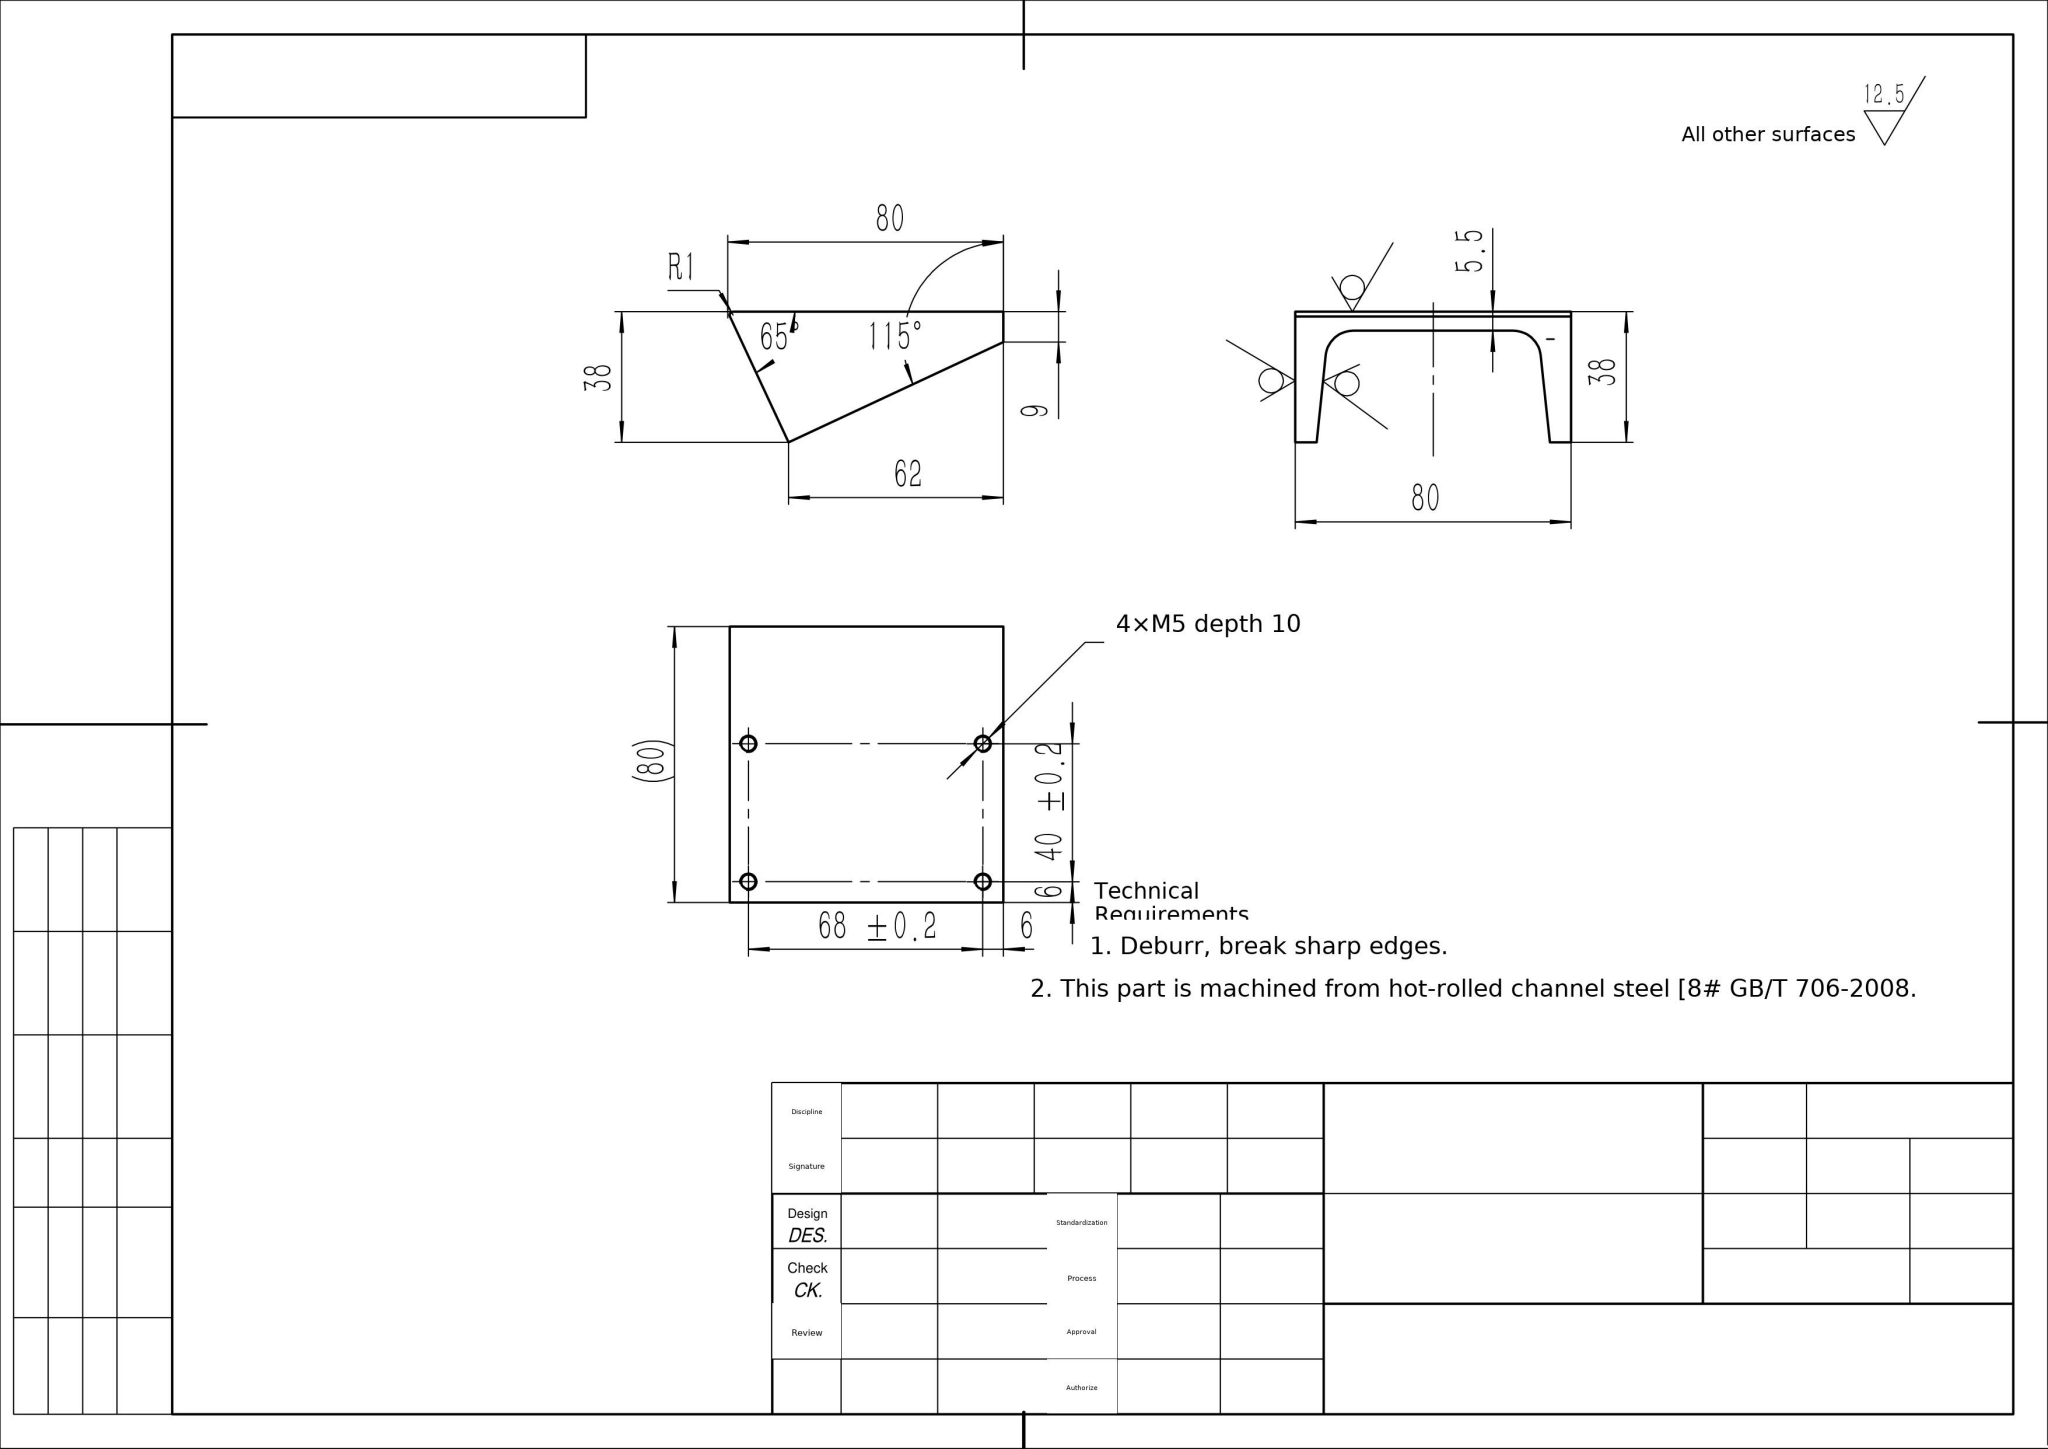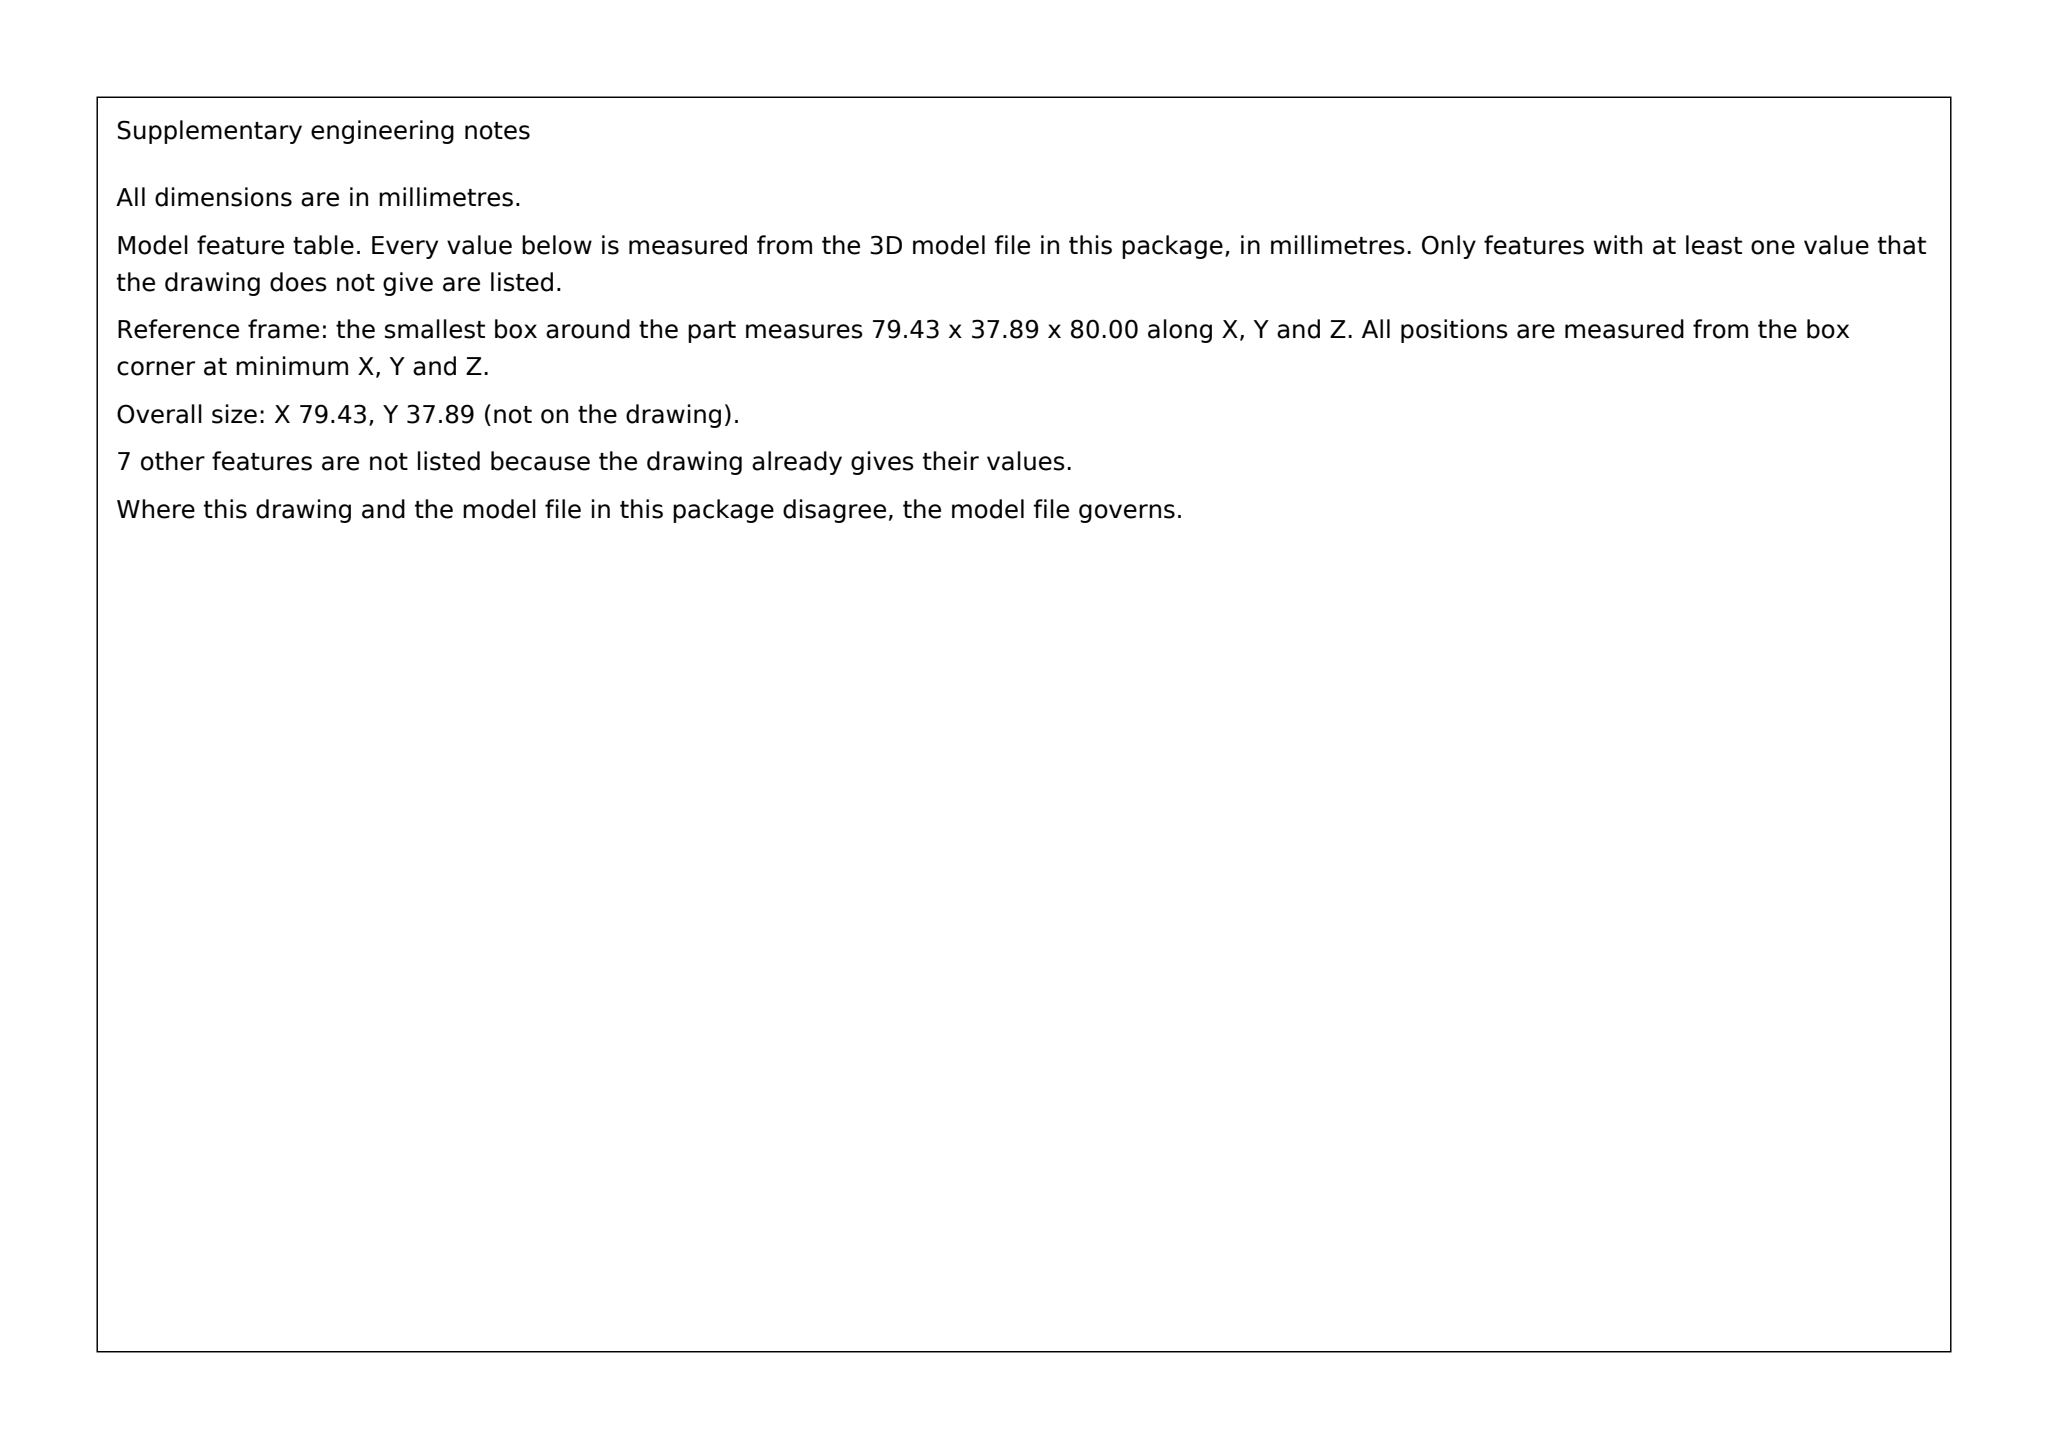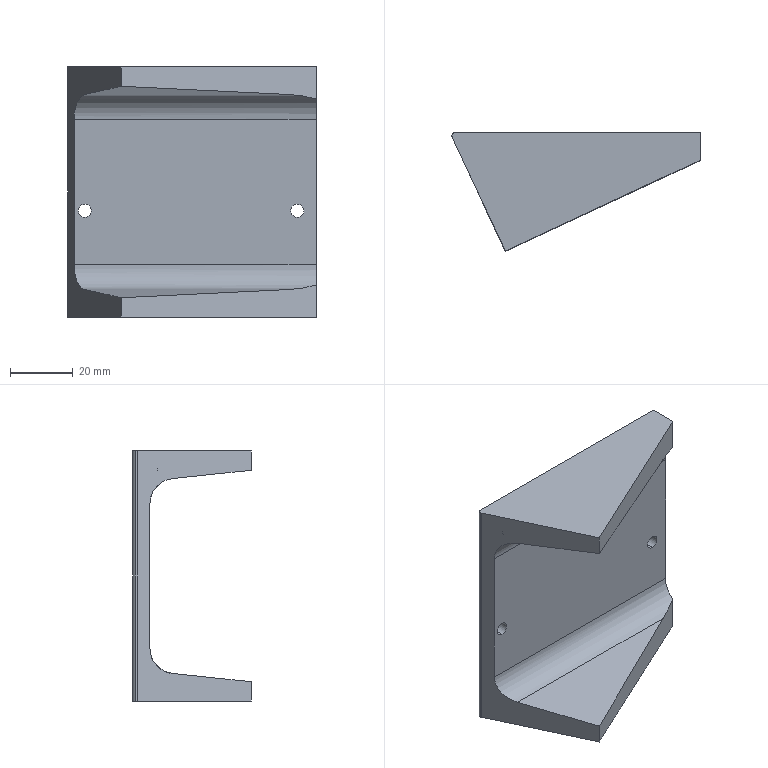Part | SolidWorks | mm | material hot-rolled channel steel [8# GB/T 706-2008 | 1 solid | 24 faces | box 79.43 x 37.89 x 80 mm | volume 58753 mm3 | cylinder 12 | plane 12 | commonest cylinder face diameters 4.2 x8 2 x2 16 x2
STEP:
#1=CARTESIAN_POINT('',(-79.43,-1.,80.));
#2=VERTEX_POINT('',#1);
#3=CARTESIAN_POINT('',(-79.337,-1.423,80.));
#4=VERTEX_POINT('',#3);
#5=CARTESIAN_POINT('',(-78.43,-1.,80.));
#6=DIRECTION('',(0.,-0.,1.));
#7=DIRECTION('',(0.,1.,0.));
#8=AXIS2_PLACEMENT_3D('',#5,#6,#7);
#9=CIRCLE('',#8,1.);
#10=EDGE_CURVE('',#2,#4,#9,.T.);
#11=ORIENTED_EDGE('',*,*,#10,.F.);
#12=CARTESIAN_POINT('',(-79.43,-1.,0.));
#13=VERTEX_POINT('',#12);
#14=CARTESIAN_POINT('',(-79.43,-1.,80.));
#15=DIRECTION('',(0.,0.,-1.));
#16=VECTOR('',#15,1000.);
#17=LINE('',#14,#16);
#18=EDGE_CURVE('',#2,#13,#17,.T.);
#19=ORIENTED_EDGE('',*,*,#18,.T.);
#20=CARTESIAN_POINT('',(-79.337,-1.423,0.));
#21=VERTEX_POINT('',#20);
#22=CARTESIAN_POINT('',(-78.43,-1.,0.));
#23=DIRECTION('',(0.,0.,-1.));
#24=DIRECTION('',(1.,0.,0.));
#25=AXIS2_PLACEMENT_3D('',#22,#23,#24);
#26=CIRCLE('',#25,1.);
#27=EDGE_CURVE('',#21,#13,#26,.T.);
#28=ORIENTED_EDGE('',*,*,#27,.F.);
#29=CARTESIAN_POINT('',(-79.337,-1.423,80.));
#30=DIRECTION('',(0.,0.,-1.));
#31=VECTOR('',#30,1000.);
#32=LINE('',#29,#31);
#33=EDGE_CURVE('',#4,#21,#32,.T.);
#34=ORIENTED_EDGE('',*,*,#33,.F.);
#35=EDGE_LOOP('',(#11,#19,#28,#34));
#36=FACE_OUTER_BOUND('',#35,.T.);
#37=CARTESIAN_POINT('',(-78.43,-1.,80.));
#38=DIRECTION('',(0.,0.,-1.));
#39=DIRECTION('',(-1.,0.,0.));
#40=AXIS2_PLACEMENT_3D('',#37,#38,#39);
#41=CYLINDRICAL_SURFACE('',#40,1.);
#42=ADVANCED_FACE('',(#36),#41,.T.);
#43=CARTESIAN_POINT('',(-6.,-5.5,31.9));
#44=VERTEX_POINT('',#43);
#45=CARTESIAN_POINT('',(-6.,-5.5,36.1));
#46=VERTEX_POINT('',#45);
#47=CARTESIAN_POINT('',(-6.,-5.5,34.));
#48=DIRECTION('',(-0.,1.,0.));
#49=DIRECTION('',(-1.,0.,0.));
#50=AXIS2_PLACEMENT_3D('',#47,#48,#49);
#51=CIRCLE('',#50,2.1);
#52=EDGE_CURVE('',#44,#46,#51,.T.);
#53=ORIENTED_EDGE('',*,*,#52,.F.);
#54=CARTESIAN_POINT('',(-6.,-0.,31.9));
#55=VERTEX_POINT('',#54);
#56=CARTESIAN_POINT('',(-6.,-0.,31.9));
#57=DIRECTION('',(0.,1.,0.));
#58=VECTOR('',#57,1000.);
#59=LINE('',#56,#58);
#60=EDGE_CURVE('',#44,#55,#59,.T.);
#61=ORIENTED_EDGE('',*,*,#60,.T.);
#62=CARTESIAN_POINT('',(-6.,-0.,36.1));
#63=VERTEX_POINT('',#62);
#64=CARTESIAN_POINT('',(-6.,-0.,34.));
#65=DIRECTION('',(0.,1.,0.));
#66=DIRECTION('',(0.,0.,1.));
#67=AXIS2_PLACEMENT_3D('',#64,#65,#66);
#68=CIRCLE('',#67,2.1);
#69=EDGE_CURVE('',#55,#63,#68,.T.);
#70=ORIENTED_EDGE('',*,*,#69,.T.);
#71=CARTESIAN_POINT('',(-6.,-0.,36.1));
#72=DIRECTION('',(0.,1.,0.));
#73=VECTOR('',#72,1000.);
#74=LINE('',#71,#73);
#75=EDGE_CURVE('',#46,#63,#74,.T.);
#76=ORIENTED_EDGE('',*,*,#75,.F.);
#77=EDGE_LOOP('',(#53,#61,#70,#76));
#78=FACE_OUTER_BOUND('',#77,.T.);
#79=CARTESIAN_POINT('',(-6.,-0.,34.));
#80=DIRECTION('',(0.,1.,0.));
#81=DIRECTION('',(0.,0.,1.));
#82=AXIS2_PLACEMENT_3D('',#79,#80,#81);
#83=CYLINDRICAL_SURFACE('',#82,2.1);
#84=ADVANCED_FACE('',(#78),#83,.F.);
#85=CARTESIAN_POINT('',(-6.,-8.,71.9));
#86=VERTEX_POINT('',#85);
#87=CARTESIAN_POINT('',(-6.,-8.,76.1));
#88=VERTEX_POINT('',#87);
#89=CARTESIAN_POINT('',(-6.,-8.,74.));
#90=DIRECTION('',(0.,1.,0.));
#91=DIRECTION('',(0.,0.,1.));
#92=AXIS2_PLACEMENT_3D('',#89,#90,#91);
#93=CIRCLE('',#92,2.1);
#94=EDGE_CURVE('',#86,#88,#93,.T.);
#95=ORIENTED_EDGE('',*,*,#94,.F.);
#96=CARTESIAN_POINT('',(-6.,-0.,71.9));
#97=VERTEX_POINT('',#96);
#98=CARTESIAN_POINT('',(-6.,-0.,71.9));
#99=DIRECTION('',(0.,1.,0.));
#100=VECTOR('',#99,1000.);
#101=LINE('',#98,#100);
#102=EDGE_CURVE('',#86,#97,#101,.T.);
#103=ORIENTED_EDGE('',*,*,#102,.T.);
#104=CARTESIAN_POINT('',(-6.,-0.,76.1));
#105=VERTEX_POINT('',#104);
#106=CARTESIAN_POINT('',(-6.,-0.,74.));
#107=DIRECTION('',(0.,1.,0.));
#108=DIRECTION('',(0.,0.,1.));
#109=AXIS2_PLACEMENT_3D('',#106,#107,#108);
#110=CIRCLE('',#109,2.1);
#111=EDGE_CURVE('',#97,#105,#110,.T.);
#112=ORIENTED_EDGE('',*,*,#111,.T.);
#113=CARTESIAN_POINT('',(-6.,-0.,76.1));
#114=DIRECTION('',(0.,1.,0.));
#115=VECTOR('',#114,1000.);
#116=LINE('',#113,#115);
#117=EDGE_CURVE('',#88,#105,#116,.T.);
#118=ORIENTED_EDGE('',*,*,#117,.F.);
#119=EDGE_LOOP('',(#95,#103,#112,#118));
#120=FACE_OUTER_BOUND('',#119,.T.);
#121=CARTESIAN_POINT('',(-6.,-0.,74.));
#122=DIRECTION('',(0.,1.,0.));
#123=DIRECTION('',(0.,0.,1.));
#124=AXIS2_PLACEMENT_3D('',#121,#122,#123);
#125=CYLINDRICAL_SURFACE('',#124,2.1);
#126=ADVANCED_FACE('',(#120),#125,.F.);
#127=CARTESIAN_POINT('',(-74.,-8.,71.9));
#128=VERTEX_POINT('',#127);
#129=CARTESIAN_POINT('',(-74.,-8.,76.1));
#130=VERTEX_POINT('',#129);
#131=CARTESIAN_POINT('',(-74.,-8.,74.));
#132=DIRECTION('',(0.,1.,0.));
#133=DIRECTION('',(0.,0.,1.));
#134=AXIS2_PLACEMENT_3D('',#131,#132,#133);
#135=CIRCLE('',#134,2.1);
#136=EDGE_CURVE('',#128,#130,#135,.T.);
#137=ORIENTED_EDGE('',*,*,#136,.F.);
#138=CARTESIAN_POINT('',(-74.,-0.,71.9));
#139=VERTEX_POINT('',#138);
#140=CARTESIAN_POINT('',(-74.,-0.,71.9));
#141=DIRECTION('',(0.,1.,0.));
#142=VECTOR('',#141,1000.);
#143=LINE('',#140,#142);
#144=EDGE_CURVE('',#128,#139,#143,.T.);
#145=ORIENTED_EDGE('',*,*,#144,.T.);
#146=CARTESIAN_POINT('',(-74.,-0.,76.1));
#147=VERTEX_POINT('',#146);
#148=CARTESIAN_POINT('',(-74.,-0.,74.));
#149=DIRECTION('',(0.,1.,0.));
#150=DIRECTION('',(0.,0.,1.));
#151=AXIS2_PLACEMENT_3D('',#148,#149,#150);
#152=CIRCLE('',#151,2.1);
#153=EDGE_CURVE('',#139,#147,#152,.T.);
#154=ORIENTED_EDGE('',*,*,#153,.T.);
#155=CARTESIAN_POINT('',(-74.,-0.,76.1));
#156=DIRECTION('',(0.,1.,0.));
#157=VECTOR('',#156,1000.);
#158=LINE('',#155,#157);
#159=EDGE_CURVE('',#130,#147,#158,.T.);
#160=ORIENTED_EDGE('',*,*,#159,.F.);
#161=EDGE_LOOP('',(#137,#145,#154,#160));
#162=FACE_OUTER_BOUND('',#161,.T.);
#163=CARTESIAN_POINT('',(-74.,-0.,74.));
#164=DIRECTION('',(0.,1.,0.));
#165=DIRECTION('',(0.,0.,1.));
#166=AXIS2_PLACEMENT_3D('',#163,#164,#165);
#167=CYLINDRICAL_SURFACE('',#166,2.1);
#168=ADVANCED_FACE('',(#162),#167,.F.);
#169=CARTESIAN_POINT('',(-74.,-5.5,31.9));
#170=VERTEX_POINT('',#169);
#171=CARTESIAN_POINT('',(-74.,-5.5,36.1));
#172=VERTEX_POINT('',#171);
#173=CARTESIAN_POINT('',(-74.,-5.5,34.));
#174=DIRECTION('',(-0.,1.,0.));
#175=DIRECTION('',(-1.,0.,0.));
#176=AXIS2_PLACEMENT_3D('',#173,#174,#175);
#177=CIRCLE('',#176,2.1);
#178=EDGE_CURVE('',#170,#172,#177,.T.);
#179=ORIENTED_EDGE('',*,*,#178,.F.);
#180=CARTESIAN_POINT('',(-74.,-0.,31.9));
#181=VERTEX_POINT('',#180);
#182=CARTESIAN_POINT('',(-74.,-0.,31.9));
#183=DIRECTION('',(0.,1.,0.));
#184=VECTOR('',#183,1000.);
#185=LINE('',#182,#184);
#186=EDGE_CURVE('',#170,#181,#185,.T.);
#187=ORIENTED_EDGE('',*,*,#186,.T.);
#188=CARTESIAN_POINT('',(-74.,-0.,36.1));
#189=VERTEX_POINT('',#188);
#190=CARTESIAN_POINT('',(-74.,-0.,34.));
#191=DIRECTION('',(0.,1.,0.));
#192=DIRECTION('',(0.,0.,1.));
#193=AXIS2_PLACEMENT_3D('',#190,#191,#192);
#194=CIRCLE('',#193,2.1);
#195=EDGE_CURVE('',#181,#189,#194,.T.);
#196=ORIENTED_EDGE('',*,*,#195,.T.);
#197=CARTESIAN_POINT('',(-74.,-0.,36.1));
#198=DIRECTION('',(0.,1.,0.));
#199=VECTOR('',#198,1000.);
#200=LINE('',#197,#199);
#201=EDGE_CURVE('',#172,#189,#200,.T.);
#202=ORIENTED_EDGE('',*,*,#201,.F.);
#203=EDGE_LOOP('',(#179,#187,#196,#202));
#204=FACE_OUTER_BOUND('',#203,.T.);
#205=CARTESIAN_POINT('',(-74.,-0.,34.));
#206=DIRECTION('',(0.,1.,0.));
#207=DIRECTION('',(0.,0.,1.));
#208=AXIS2_PLACEMENT_3D('',#205,#206,#207);
#209=CYLINDRICAL_SURFACE('',#208,2.1);
#210=ADVANCED_FACE('',(#204),#209,.F.);
#211=CARTESIAN_POINT('',(-78.43,-0.,80.));
#212=VERTEX_POINT('',#211);
#213=CARTESIAN_POINT('',(0.,0.,80.));
#214=VERTEX_POINT('',#213);
#215=CARTESIAN_POINT('',(-80.,-0.,80.));
#216=DIRECTION('',(1.,0.,0.));
#217=VECTOR('',#216,1000.);
#218=LINE('',#215,#217);
#219=EDGE_CURVE('',#212,#214,#218,.T.);
#220=ORIENTED_EDGE('',*,*,#219,.F.);
#221=CARTESIAN_POINT('',(-78.43,-1.,80.));
#222=DIRECTION('',(0.,-0.,1.));
#223=DIRECTION('',(0.,1.,0.));
#224=AXIS2_PLACEMENT_3D('',#221,#222,#223);
#225=CIRCLE('',#224,1.);
#226=EDGE_CURVE('',#212,#2,#225,.T.);
#227=ORIENTED_EDGE('',*,*,#226,.T.);
#228=ORIENTED_EDGE('',*,*,#10,.T.);
#229=CARTESIAN_POINT('',(-62.331,-37.892,80.));
#230=VERTEX_POINT('',#229);
#231=CARTESIAN_POINT('',(-65.712,-30.642,80.));
#232=DIRECTION('',(0.4226,-0.9063,0.));
#233=VECTOR('',#232,1000.);
#234=LINE('',#231,#233);
#235=EDGE_CURVE('',#4,#230,#234,.T.);
#236=ORIENTED_EDGE('',*,*,#235,.T.);
#237=CARTESIAN_POINT('',(-0.,-8.827,80.));
#238=VERTEX_POINT('',#237);
#239=CARTESIAN_POINT('',(-0.,-8.827,80.));
#240=DIRECTION('',(0.9063,0.4226,0.));
#241=VECTOR('',#240,1000.);
#242=LINE('',#239,#241);
#243=EDGE_CURVE('',#230,#238,#242,.T.);
#244=ORIENTED_EDGE('',*,*,#243,.T.);
#245=CARTESIAN_POINT('',(0.,-45.,80.));
#246=DIRECTION('',(-0.,1.,0.));
#247=VECTOR('',#246,1000.);
#248=LINE('',#245,#247);
#249=EDGE_CURVE('',#238,#214,#248,.T.);
#250=ORIENTED_EDGE('',*,*,#249,.T.);
#251=EDGE_LOOP('',(#220,#227,#228,#236,#244,#250));
#252=FACE_OUTER_BOUND('',#251,.T.);
#253=CARTESIAN_POINT('',(-80.,-45.,80.));
#254=DIRECTION('',(-0.,0.,-1.));
#255=DIRECTION('',(0.,1.,0.));
#256=AXIS2_PLACEMENT_3D('',#253,#254,#255);
#257=PLANE('',#256);
#258=ADVANCED_FACE('',(#252),#257,.F.);
#259=CARTESIAN_POINT('',(-6.,-0.,34.));
#260=DIRECTION('',(0.,1.,0.));
#261=DIRECTION('',(0.,0.,1.));
#262=AXIS2_PLACEMENT_3D('',#259,#260,#261);
#263=CIRCLE('',#262,2.1);
#264=EDGE_CURVE('',#63,#55,#263,.T.);
#265=ORIENTED_EDGE('',*,*,#264,.F.);
#266=ORIENTED_EDGE('',*,*,#69,.F.);
#267=EDGE_LOOP('',(#265,#266));
#268=FACE_BOUND('',#267,.T.);
#269=CARTESIAN_POINT('',(-6.,-0.,74.));
#270=DIRECTION('',(0.,1.,0.));
#271=DIRECTION('',(0.,0.,1.));
#272=AXIS2_PLACEMENT_3D('',#269,#270,#271);
#273=CIRCLE('',#272,2.1);
#274=EDGE_CURVE('',#105,#97,#273,.T.);
#275=ORIENTED_EDGE('',*,*,#274,.F.);
#276=ORIENTED_EDGE('',*,*,#111,.F.);
#277=EDGE_LOOP('',(#275,#276));
#278=FACE_BOUND('',#277,.T.);
#279=CARTESIAN_POINT('',(-74.,-0.,74.));
#280=DIRECTION('',(0.,1.,0.));
#281=DIRECTION('',(0.,0.,1.));
#282=AXIS2_PLACEMENT_3D('',#279,#280,#281);
#283=CIRCLE('',#282,2.1);
#284=EDGE_CURVE('',#147,#139,#283,.T.);
#285=ORIENTED_EDGE('',*,*,#284,.F.);
#286=ORIENTED_EDGE('',*,*,#153,.F.);
#287=EDGE_LOOP('',(#285,#286));
#288=FACE_BOUND('',#287,.T.);
#289=CARTESIAN_POINT('',(-74.,-0.,34.));
#290=DIRECTION('',(0.,1.,0.));
#291=DIRECTION('',(0.,0.,1.));
#292=AXIS2_PLACEMENT_3D('',#289,#290,#291);
#293=CIRCLE('',#292,2.1);
#294=EDGE_CURVE('',#189,#181,#293,.T.);
#295=ORIENTED_EDGE('',*,*,#294,.F.);
#296=ORIENTED_EDGE('',*,*,#195,.F.);
#297=EDGE_LOOP('',(#295,#296));
#298=FACE_BOUND('',#297,.T.);
#299=CARTESIAN_POINT('',(-78.43,-0.,0.));
#300=VERTEX_POINT('',#299);
#301=CARTESIAN_POINT('',(0.,0.,0.));
#302=VERTEX_POINT('',#301);
#303=CARTESIAN_POINT('',(-80.,-0.,0.));
#304=DIRECTION('',(1.,0.,0.));
#305=VECTOR('',#304,1000.);
#306=LINE('',#303,#305);
#307=EDGE_CURVE('',#300,#302,#306,.T.);
#308=ORIENTED_EDGE('',*,*,#307,.F.);
#309=CARTESIAN_POINT('',(-78.43,-0.,80.));
#310=DIRECTION('',(0.,0.,1.));
#311=VECTOR('',#310,1000.);
#312=LINE('',#309,#311);
#313=EDGE_CURVE('',#300,#212,#312,.T.);
#314=ORIENTED_EDGE('',*,*,#313,.T.);
#315=ORIENTED_EDGE('',*,*,#219,.T.);
#316=CARTESIAN_POINT('',(0.,0.,80.));
#317=DIRECTION('',(0.,0.,-1.));
#318=VECTOR('',#317,1000.);
#319=LINE('',#316,#318);
#320=EDGE_CURVE('',#214,#302,#319,.T.);
#321=ORIENTED_EDGE('',*,*,#320,.T.);
#322=EDGE_LOOP('',(#308,#314,#315,#321));
#323=FACE_OUTER_BOUND('',#322,.T.);
#324=CARTESIAN_POINT('',(-80.,-0.,80.));
#325=DIRECTION('',(0.,-1.,0.));
#326=DIRECTION('',(1.,0.,0.));
#327=AXIS2_PLACEMENT_3D('',#324,#325,#326);
#328=PLANE('',#327);
#329=ADVANCED_FACE('',(#268,#278,#288,#298,#323),#328,.F.);
#330=CARTESIAN_POINT('',(-62.331,-37.892,0.));
#331=VERTEX_POINT('',#330);
#332=CARTESIAN_POINT('',(-65.712,-30.642,0.));
#333=DIRECTION('',(0.4226,-0.9063,0.));
#334=VECTOR('',#333,1000.);
#335=LINE('',#332,#334);
#336=EDGE_CURVE('',#21,#331,#335,.T.);
#337=ORIENTED_EDGE('',*,*,#336,.F.);
#338=ORIENTED_EDGE('',*,*,#27,.T.);
#339=CARTESIAN_POINT('',(-78.43,-1.,0.));
#340=DIRECTION('',(0.,0.,-1.));
#341=DIRECTION('',(1.,0.,0.));
#342=AXIS2_PLACEMENT_3D('',#339,#340,#341);
#343=CIRCLE('',#342,1.);
#344=EDGE_CURVE('',#13,#300,#343,.T.);
#345=ORIENTED_EDGE('',*,*,#344,.T.);
#346=ORIENTED_EDGE('',*,*,#307,.T.);
#347=CARTESIAN_POINT('',(0.,-8.827,0.));
#348=VERTEX_POINT('',#347);
#349=CARTESIAN_POINT('',(0.,-45.,0.));
#350=DIRECTION('',(0.,-1.,0.));
#351=VECTOR('',#350,1000.);
#352=LINE('',#349,#351);
#353=EDGE_CURVE('',#302,#348,#352,.T.);
#354=ORIENTED_EDGE('',*,*,#353,.T.);
#355=CARTESIAN_POINT('',(-0.,-8.827,0.));
#356=DIRECTION('',(0.9063,0.4226,0.));
#357=VECTOR('',#356,1000.);
#358=LINE('',#355,#357);
#359=EDGE_CURVE('',#331,#348,#358,.T.);
#360=ORIENTED_EDGE('',*,*,#359,.F.);
#361=EDGE_LOOP('',(#337,#338,#345,#346,#354,#360));
#362=FACE_OUTER_BOUND('',#361,.T.);
#363=CARTESIAN_POINT('',(-80.,-45.,0.));
#364=DIRECTION('',(0.,0.,1.));
#365=DIRECTION('',(1.,0.,0.));
#366=AXIS2_PLACEMENT_3D('',#363,#364,#365);
#367=PLANE('',#366);
#368=ADVANCED_FACE('',(#362),#367,.F.);
#369=CARTESIAN_POINT('',(-74.095,-12.664,8.823));
#370=VERTEX_POINT('',#369);
#371=CARTESIAN_POINT('',(-8.228,-12.664,8.823));
#372=VERTEX_POINT('',#371);
#373=CARTESIAN_POINT('',(-80.,-12.664,8.823));
#374=DIRECTION('',(1.,0.,0.));
#375=VECTOR('',#374,1000.);
#376=LINE('',#373,#375);
#377=EDGE_CURVE('',#370,#372,#376,.T.);
#378=ORIENTED_EDGE('',*,*,#377,.F.);
#379=CARTESIAN_POINT('',(-62.331,-37.892,6.171));
#380=VERTEX_POINT('',#379);
#381=CARTESIAN_POINT('',(-75.14,-10.422,9.058));
#382=DIRECTION('',(0.4207,-0.9022,-0.09483));
#383=VECTOR('',#382,1000.);
#384=LINE('',#381,#383);
#385=EDGE_CURVE('',#370,#380,#384,.T.);
#386=ORIENTED_EDGE('',*,*,#385,.T.);
#387=CARTESIAN_POINT('',(-67.065,-40.1,5.939));
#388=DIRECTION('',(0.9054,0.4222,0.04438));
#389=VECTOR('',#388,1000.);
#390=LINE('',#387,#389);
#391=EDGE_CURVE('',#380,#372,#390,.T.);
#392=ORIENTED_EDGE('',*,*,#391,.T.);
#393=EDGE_LOOP('',(#378,#386,#392));
#394=FACE_OUTER_BOUND('',#393,.T.);
#395=CARTESIAN_POINT('',(-80.,-12.664,8.823));
#396=DIRECTION('',(-0.,0.1045,-0.9945));
#397=DIRECTION('',(0.,0.9945,0.1045));
#398=AXIS2_PLACEMENT_3D('',#395,#396,#397);
#399=PLANE('',#398);
#400=ADVANCED_FACE('',(#394),#399,.F.);
#401=CARTESIAN_POINT('',(-77.435,-5.5,16.779));
#402=VERTEX_POINT('',#401);
#403=CARTESIAN_POINT('',(0.,-5.5,16.779));
#404=VERTEX_POINT('',#403);
#405=CARTESIAN_POINT('',(-80.,-5.5,16.779));
#406=DIRECTION('',(1.,0.,0.));
#407=VECTOR('',#406,1000.);
#408=LINE('',#405,#407);
#409=EDGE_CURVE('',#402,#404,#408,.T.);
#410=ORIENTED_EDGE('',*,*,#409,.F.);
#411=CARTESIAN_POINT('',(-77.435,-5.5,16.779));
#412=CARTESIAN_POINT('',(-77.435,-5.5,12.473));
#413=CARTESIAN_POINT('',(-76.092,-8.381,9.273));
#414=CARTESIAN_POINT('',(-74.095,-12.664,8.823));
#415=(BOUNDED_CURVE()B_SPLINE_CURVE(3,(#411,#412,#413,#414),.UNSPECIFIED.,.F.,.F.)B_SPLINE_CURVE_WITH_KNOTS((4,4),(3.142,4.608),.UNSPECIFIED.)CURVE()GEOMETRIC_REPRESENTATION_ITEM()RATIONAL_B_SPLINE_CURVE((1.,0.8288,0.8288,1.))REPRESENTATION_ITEM(''));
#416=EDGE_CURVE('',#402,#370,#415,.T.);
#417=ORIENTED_EDGE('',*,*,#416,.T.);
#418=ORIENTED_EDGE('',*,*,#377,.T.);
#419=CARTESIAN_POINT('',(-0.,-8.827,10.286));
#420=VERTEX_POINT('',#419);
#421=CARTESIAN_POINT('',(-8.228,-12.664,8.823));
#422=CARTESIAN_POINT('',(-5.242,-11.271,8.969));
#423=CARTESIAN_POINT('',(-2.437,-9.963,9.468));
#424=CARTESIAN_POINT('',(-0.,-8.827,10.286));
#425=(BOUNDED_CURVE()B_SPLINE_CURVE(3,(#421,#422,#423,#424),.UNSPECIFIED.,.F.,.F.)B_SPLINE_CURVE_WITH_KNOTS((4,4),(4.817,5.336),.UNSPECIFIED.)CURVE()GEOMETRIC_REPRESENTATION_ITEM()RATIONAL_B_SPLINE_CURVE((1.,0.9777,0.9777,1.))REPRESENTATION_ITEM(''));
#426=EDGE_CURVE('',#372,#420,#425,.T.);
#427=ORIENTED_EDGE('',*,*,#426,.T.);
#428=CARTESIAN_POINT('',(0.,-13.5,16.779));
#429=DIRECTION('',(1.,0.,0.));
#430=DIRECTION('',(0.,-1.,0.));
#431=AXIS2_PLACEMENT_3D('',#428,#429,#430);
#432=CIRCLE('',#431,8.);
#433=EDGE_CURVE('',#420,#404,#432,.T.);
#434=ORIENTED_EDGE('',*,*,#433,.T.);
#435=EDGE_LOOP('',(#410,#417,#418,#427,#434));
#436=FACE_OUTER_BOUND('',#435,.T.);
#437=CARTESIAN_POINT('',(-80.,-13.5,16.779));
#438=DIRECTION('',(1.,0.,0.));
#439=DIRECTION('',(0.,1.,0.));
#440=AXIS2_PLACEMENT_3D('',#437,#438,#439);
#441=CYLINDRICAL_SURFACE('',#440,8.);
#442=ADVANCED_FACE('',(#436),#441,.F.);
#443=CARTESIAN_POINT('',(-6.,-5.5,34.));
#444=DIRECTION('',(-0.,1.,0.));
#445=DIRECTION('',(-1.,0.,0.));
#446=AXIS2_PLACEMENT_3D('',#443,#444,#445);
#447=CIRCLE('',#446,2.1);
#448=EDGE_CURVE('',#46,#44,#447,.T.);
#449=ORIENTED_EDGE('',*,*,#448,.T.);
#450=ORIENTED_EDGE('',*,*,#52,.T.);
#451=EDGE_LOOP('',(#449,#450));
#452=FACE_BOUND('',#451,.T.);
#453=CARTESIAN_POINT('',(-74.,-5.5,34.));
#454=DIRECTION('',(-0.,1.,0.));
#455=DIRECTION('',(-1.,0.,0.));
#456=AXIS2_PLACEMENT_3D('',#453,#454,#455);
#457=CIRCLE('',#456,2.1);
#458=EDGE_CURVE('',#172,#170,#457,.T.);
#459=ORIENTED_EDGE('',*,*,#458,.T.);
#460=ORIENTED_EDGE('',*,*,#178,.T.);
#461=EDGE_LOOP('',(#459,#460));
#462=FACE_BOUND('',#461,.T.);
#463=CARTESIAN_POINT('',(-77.435,-5.5,63.221));
#464=VERTEX_POINT('',#463);
#465=CARTESIAN_POINT('',(0.,-5.5,63.221));
#466=VERTEX_POINT('',#465);
#467=CARTESIAN_POINT('',(-80.,-5.5,63.221));
#468=DIRECTION('',(1.,0.,0.));
#469=VECTOR('',#468,1000.);
#470=LINE('',#467,#469);
#471=EDGE_CURVE('',#464,#466,#470,.T.);
#472=ORIENTED_EDGE('',*,*,#471,.F.);
#473=CARTESIAN_POINT('',(-77.435,-5.5,63.221));
#474=DIRECTION('',(0.,0.,-1.));
#475=VECTOR('',#474,1000.);
#476=LINE('',#473,#475);
#477=EDGE_CURVE('',#464,#402,#476,.T.);
#478=ORIENTED_EDGE('',*,*,#477,.T.);
#479=ORIENTED_EDGE('',*,*,#409,.T.);
#480=CARTESIAN_POINT('',(0.,-5.5,63.221));
#481=DIRECTION('',(0.,0.,1.));
#482=VECTOR('',#481,1000.);
#483=LINE('',#480,#482);
#484=EDGE_CURVE('',#404,#466,#483,.T.);
#485=ORIENTED_EDGE('',*,*,#484,.T.);
#486=EDGE_LOOP('',(#472,#478,#479,#485));
#487=FACE_OUTER_BOUND('',#486,.T.);
#488=CARTESIAN_POINT('',(-80.,-5.5,63.221));
#489=DIRECTION('',(-0.,1.,0.));
#490=DIRECTION('',(-1.,-0.,0.));
#491=AXIS2_PLACEMENT_3D('',#488,#489,#490);
#492=PLANE('',#491);
#493=ADVANCED_FACE('',(#452,#462,#487),#492,.F.);
#494=CARTESIAN_POINT('',(-74.095,-12.664,71.177));
#495=VERTEX_POINT('',#494);
#496=CARTESIAN_POINT('',(-8.228,-12.664,71.177));
#497=VERTEX_POINT('',#496);
#498=CARTESIAN_POINT('',(-80.,-12.664,71.177));
#499=DIRECTION('',(1.,0.,0.));
#500=VECTOR('',#499,1000.);
#501=LINE('',#498,#500);
#502=EDGE_CURVE('',#495,#497,#501,.T.);
#503=ORIENTED_EDGE('',*,*,#502,.F.);
#504=CARTESIAN_POINT('',(-74.095,-12.664,71.177));
#505=CARTESIAN_POINT('',(-76.092,-8.381,70.727));
#506=CARTESIAN_POINT('',(-77.435,-5.5,67.527));
#507=CARTESIAN_POINT('',(-77.435,-5.5,63.221));
#508=(BOUNDED_CURVE()B_SPLINE_CURVE(3,(#504,#505,#506,#507),.UNSPECIFIED.,.F.,.F.)B_SPLINE_CURVE_WITH_KNOTS((4,4),(1.676,3.142),.UNSPECIFIED.)CURVE()GEOMETRIC_REPRESENTATION_ITEM()RATIONAL_B_SPLINE_CURVE((1.,0.8288,0.8288,1.))REPRESENTATION_ITEM(''));
#509=EDGE_CURVE('',#495,#464,#508,.T.);
#510=ORIENTED_EDGE('',*,*,#509,.T.);
#511=ORIENTED_EDGE('',*,*,#471,.T.);
#512=CARTESIAN_POINT('',(0.,-8.827,69.714));
#513=VERTEX_POINT('',#512);
#514=CARTESIAN_POINT('',(0.,-13.5,63.221));
#515=DIRECTION('',(1.,0.,0.));
#516=DIRECTION('',(-0.,1.,0.));
#517=AXIS2_PLACEMENT_3D('',#514,#515,#516);
#518=CIRCLE('',#517,8.);
#519=EDGE_CURVE('',#466,#513,#518,.T.);
#520=ORIENTED_EDGE('',*,*,#519,.T.);
#521=CARTESIAN_POINT('',(0.,-8.827,69.714));
#522=CARTESIAN_POINT('',(-2.437,-9.963,70.532));
#523=CARTESIAN_POINT('',(-5.242,-11.271,71.031));
#524=CARTESIAN_POINT('',(-8.228,-12.664,71.177));
#525=(BOUNDED_CURVE()B_SPLINE_CURVE(3,(#521,#522,#523,#524),.UNSPECIFIED.,.F.,.F.)B_SPLINE_CURVE_WITH_KNOTS((4,4),(0.947,1.466),.UNSPECIFIED.)CURVE()GEOMETRIC_REPRESENTATION_ITEM()RATIONAL_B_SPLINE_CURVE((1.,0.9777,0.9777,1.))REPRESENTATION_ITEM(''));
#526=EDGE_CURVE('',#513,#497,#525,.T.);
#527=ORIENTED_EDGE('',*,*,#526,.T.);
#528=EDGE_LOOP('',(#503,#510,#511,#520,#527));
#529=FACE_OUTER_BOUND('',#528,.T.);
#530=CARTESIAN_POINT('',(-80.,-13.5,63.221));
#531=DIRECTION('',(1.,0.,0.));
#532=DIRECTION('',(0.,1.,0.));
#533=AXIS2_PLACEMENT_3D('',#530,#531,#532);
#534=CYLINDRICAL_SURFACE('',#533,8.);
#535=ADVANCED_FACE('',(#529),#534,.F.);
#536=CARTESIAN_POINT('',(-62.331,-37.892,73.829));
#537=VERTEX_POINT('',#536);
#538=CARTESIAN_POINT('',(-67.065,-40.1,74.061));
#539=DIRECTION('',(-0.9054,-0.4222,0.04438));
#540=VECTOR('',#539,1000.);
#541=LINE('',#538,#540);
#542=EDGE_CURVE('',#497,#537,#541,.T.);
#543=ORIENTED_EDGE('',*,*,#542,.T.);
#544=CARTESIAN_POINT('',(-75.14,-10.422,70.942));
#545=DIRECTION('',(-0.4207,0.9022,-0.09483));
#546=VECTOR('',#545,1000.);
#547=LINE('',#544,#546);
#548=EDGE_CURVE('',#537,#495,#547,.T.);
#549=ORIENTED_EDGE('',*,*,#548,.T.);
#550=ORIENTED_EDGE('',*,*,#502,.T.);
#551=EDGE_LOOP('',(#543,#549,#550));
#552=FACE_OUTER_BOUND('',#551,.T.);
#553=CARTESIAN_POINT('',(-80.,-12.664,71.177));
#554=DIRECTION('',(-0.,0.1045,0.9945));
#555=DIRECTION('',(0.,-0.9945,0.1045));
#556=AXIS2_PLACEMENT_3D('',#553,#554,#555);
#557=PLANE('',#556);
#558=ADVANCED_FACE('',(#552),#557,.F.);
#559=ORIENTED_EDGE('',*,*,#249,.F.);
#560=CARTESIAN_POINT('',(-0.,-8.827,80.));
#561=DIRECTION('',(0.,0.,-1.));
#562=VECTOR('',#561,1000.);
#563=LINE('',#560,#562);
#564=EDGE_CURVE('',#238,#513,#563,.T.);
#565=ORIENTED_EDGE('',*,*,#564,.T.);
#566=ORIENTED_EDGE('',*,*,#519,.F.);
#567=ORIENTED_EDGE('',*,*,#484,.F.);
#568=ORIENTED_EDGE('',*,*,#433,.F.);
#569=CARTESIAN_POINT('',(0.,-8.827,78.177));
#570=DIRECTION('',(0.,0.,-1.));
#571=VECTOR('',#570,1000.);
#572=LINE('',#569,#571);
#573=EDGE_CURVE('',#420,#348,#572,.T.);
#574=ORIENTED_EDGE('',*,*,#573,.T.);
#575=ORIENTED_EDGE('',*,*,#353,.F.);
#576=ORIENTED_EDGE('',*,*,#320,.F.);
#577=EDGE_LOOP('',(#559,#565,#566,#567,#568,#574,#575,#576));
#578=FACE_OUTER_BOUND('',#577,.T.);
#579=CARTESIAN_POINT('',(0.,-41.,78.177));
#580=DIRECTION('',(-1.,-0.,0.));
#581=DIRECTION('',(0.,-1.,0.));
#582=AXIS2_PLACEMENT_3D('',#579,#580,#581);
#583=PLANE('',#582);
#584=ADVANCED_FACE('',(#578),#583,.F.);
#585=ORIENTED_EDGE('',*,*,#186,.F.);
#586=ORIENTED_EDGE('',*,*,#458,.F.);
#587=ORIENTED_EDGE('',*,*,#201,.T.);
#588=ORIENTED_EDGE('',*,*,#294,.T.);
#589=EDGE_LOOP('',(#585,#586,#587,#588));
#590=FACE_OUTER_BOUND('',#589,.T.);
#591=CARTESIAN_POINT('',(-74.,-0.,34.));
#592=DIRECTION('',(0.,1.,0.));
#593=DIRECTION('',(0.,0.,1.));
#594=AXIS2_PLACEMENT_3D('',#591,#592,#593);
#595=CYLINDRICAL_SURFACE('',#594,2.1);
#596=ADVANCED_FACE('',(#590),#595,.F.);
#597=CARTESIAN_POINT('',(-74.,-8.,74.));
#598=DIRECTION('',(0.,1.,0.));
#599=DIRECTION('',(0.,0.,1.));
#600=AXIS2_PLACEMENT_3D('',#597,#598,#599);
#601=CIRCLE('',#600,2.1);
#602=EDGE_CURVE('',#130,#128,#601,.T.);
#603=ORIENTED_EDGE('',*,*,#602,.T.);
#604=ORIENTED_EDGE('',*,*,#136,.T.);
#605=EDGE_LOOP('',(#603,#604));
#606=FACE_OUTER_BOUND('',#605,.T.);
#607=CARTESIAN_POINT('',(-74.,-8.,74.));
#608=DIRECTION('',(0.,-1.,0.));
#609=DIRECTION('',(0.,0.,-1.));
#610=AXIS2_PLACEMENT_3D('',#607,#608,#609);
#611=PLANE('',#610);
#612=ADVANCED_FACE('',(#606),#611,.F.);
#613=ORIENTED_EDGE('',*,*,#144,.F.);
#614=ORIENTED_EDGE('',*,*,#602,.F.);
#615=ORIENTED_EDGE('',*,*,#159,.T.);
#616=ORIENTED_EDGE('',*,*,#284,.T.);
#617=EDGE_LOOP('',(#613,#614,#615,#616));
#618=FACE_OUTER_BOUND('',#617,.T.);
#619=CARTESIAN_POINT('',(-74.,-0.,74.));
#620=DIRECTION('',(0.,1.,0.));
#621=DIRECTION('',(0.,0.,1.));
#622=AXIS2_PLACEMENT_3D('',#619,#620,#621);
#623=CYLINDRICAL_SURFACE('',#622,2.1);
#624=ADVANCED_FACE('',(#618),#623,.F.);
#625=CARTESIAN_POINT('',(-6.,-8.,74.));
#626=DIRECTION('',(0.,1.,0.));
#627=DIRECTION('',(0.,0.,1.));
#628=AXIS2_PLACEMENT_3D('',#625,#626,#627);
#629=CIRCLE('',#628,2.1);
#630=EDGE_CURVE('',#88,#86,#629,.T.);
#631=ORIENTED_EDGE('',*,*,#630,.T.);
#632=ORIENTED_EDGE('',*,*,#94,.T.);
#633=EDGE_LOOP('',(#631,#632));
#634=FACE_OUTER_BOUND('',#633,.T.);
#635=CARTESIAN_POINT('',(-6.,-8.,74.));
#636=DIRECTION('',(0.,-1.,0.));
#637=DIRECTION('',(0.,0.,-1.));
#638=AXIS2_PLACEMENT_3D('',#635,#636,#637);
#639=PLANE('',#638);
#640=ADVANCED_FACE('',(#634),#639,.F.);
#641=ORIENTED_EDGE('',*,*,#102,.F.);
#642=ORIENTED_EDGE('',*,*,#630,.F.);
#643=ORIENTED_EDGE('',*,*,#117,.T.);
#644=ORIENTED_EDGE('',*,*,#274,.T.);
#645=EDGE_LOOP('',(#641,#642,#643,#644));
#646=FACE_OUTER_BOUND('',#645,.T.);
#647=CARTESIAN_POINT('',(-6.,-0.,74.));
#648=DIRECTION('',(0.,1.,0.));
#649=DIRECTION('',(0.,0.,1.));
#650=AXIS2_PLACEMENT_3D('',#647,#648,#649);
#651=CYLINDRICAL_SURFACE('',#650,2.1);
#652=ADVANCED_FACE('',(#646),#651,.F.);
#653=ORIENTED_EDGE('',*,*,#60,.F.);
#654=ORIENTED_EDGE('',*,*,#448,.F.);
#655=ORIENTED_EDGE('',*,*,#75,.T.);
#656=ORIENTED_EDGE('',*,*,#264,.T.);
#657=EDGE_LOOP('',(#653,#654,#655,#656));
#658=FACE_OUTER_BOUND('',#657,.T.);
#659=CARTESIAN_POINT('',(-6.,-0.,34.));
#660=DIRECTION('',(0.,1.,0.));
#661=DIRECTION('',(0.,0.,1.));
#662=AXIS2_PLACEMENT_3D('',#659,#660,#661);
#663=CYLINDRICAL_SURFACE('',#662,2.1);
#664=ADVANCED_FACE('',(#658),#663,.F.);
#665=ORIENTED_EDGE('',*,*,#391,.F.);
#666=CARTESIAN_POINT('',(-62.331,-37.892,80.));
#667=DIRECTION('',(0.,0.,-1.));
#668=VECTOR('',#667,1000.);
#669=LINE('',#666,#668);
#670=EDGE_CURVE('',#380,#331,#669,.T.);
#671=ORIENTED_EDGE('',*,*,#670,.T.);
#672=ORIENTED_EDGE('',*,*,#359,.T.);
#673=ORIENTED_EDGE('',*,*,#573,.F.);
#674=ORIENTED_EDGE('',*,*,#426,.F.);
#675=EDGE_LOOP('',(#665,#671,#672,#673,#674));
#676=FACE_OUTER_BOUND('',#675,.T.);
#677=CARTESIAN_POINT('',(-0.,-8.827,80.));
#678=DIRECTION('',(-0.4226,0.9063,0.));
#679=DIRECTION('',(-0.9063,-0.4226,0.));
#680=AXIS2_PLACEMENT_3D('',#677,#678,#679);
#681=PLANE('',#680);
#682=ADVANCED_FACE('',(#676),#681,.F.);
#683=ORIENTED_EDGE('',*,*,#243,.F.);
#684=CARTESIAN_POINT('',(-62.331,-37.892,80.));
#685=DIRECTION('',(0.,0.,-1.));
#686=VECTOR('',#685,1000.);
#687=LINE('',#684,#686);
#688=EDGE_CURVE('',#230,#537,#687,.T.);
#689=ORIENTED_EDGE('',*,*,#688,.T.);
#690=ORIENTED_EDGE('',*,*,#542,.F.);
#691=ORIENTED_EDGE('',*,*,#526,.F.);
#692=ORIENTED_EDGE('',*,*,#564,.F.);
#693=EDGE_LOOP('',(#683,#689,#690,#691,#692));
#694=FACE_OUTER_BOUND('',#693,.T.);
#695=CARTESIAN_POINT('',(-0.,-8.827,80.));
#696=DIRECTION('',(-0.4226,0.9063,0.));
#697=DIRECTION('',(-0.9063,-0.4226,0.));
#698=AXIS2_PLACEMENT_3D('',#695,#696,#697);
#699=PLANE('',#698);
#700=ADVANCED_FACE('',(#694),#699,.F.);
#701=ORIENTED_EDGE('',*,*,#235,.F.);
#702=ORIENTED_EDGE('',*,*,#33,.T.);
#703=ORIENTED_EDGE('',*,*,#336,.T.);
#704=ORIENTED_EDGE('',*,*,#670,.F.);
#705=ORIENTED_EDGE('',*,*,#385,.F.);
#706=ORIENTED_EDGE('',*,*,#416,.F.);
#707=ORIENTED_EDGE('',*,*,#477,.F.);
#708=ORIENTED_EDGE('',*,*,#509,.F.);
#709=ORIENTED_EDGE('',*,*,#548,.F.);
#710=ORIENTED_EDGE('',*,*,#688,.F.);
#711=EDGE_LOOP('',(#701,#702,#703,#704,#705,#706,#707,#708,#709,#710));
#712=FACE_OUTER_BOUND('',#711,.T.);
#713=CARTESIAN_POINT('',(-65.712,-30.642,80.));
#714=DIRECTION('',(0.9063,0.4226,0.));
#715=DIRECTION('',(-0.4226,0.9063,0.));
#716=AXIS2_PLACEMENT_3D('',#713,#714,#715);
#717=PLANE('',#716);
#718=ADVANCED_FACE('',(#712),#717,.F.);
#719=ORIENTED_EDGE('',*,*,#18,.F.);
#720=ORIENTED_EDGE('',*,*,#226,.F.);
#721=ORIENTED_EDGE('',*,*,#313,.F.);
#722=ORIENTED_EDGE('',*,*,#344,.F.);
#723=EDGE_LOOP('',(#719,#720,#721,#722));
#724=FACE_OUTER_BOUND('',#723,.T.);
#725=CARTESIAN_POINT('',(-78.43,-1.,80.));
#726=DIRECTION('',(0.,0.,-1.));
#727=DIRECTION('',(-1.,0.,0.));
#728=AXIS2_PLACEMENT_3D('',#725,#726,#727);
#729=CYLINDRICAL_SURFACE('',#728,1.);
#730=ADVANCED_FACE('',(#724),#729,.T.);
#731=CLOSED_SHELL('',(#42,#84,#126,#168,#210,#258,#329,#368,#400,#442,#493,#535,#558,#584,#596,#612,#624,#640,#652,#664,#682,#700,#718,#730));
#732=MANIFOLD_SOLID_BREP('',#731);
#733=CARTESIAN_POINT('',(0.,0.,0.));
#734=DIRECTION('',(0.,0.,1.));
#735=DIRECTION('',(1.,0.,0.));
#736=AXIS2_PLACEMENT_3D('',#733,#734,#735);
#737=(LENGTH_UNIT()NAMED_UNIT(*)SI_UNIT(.MILLI.,.METRE.));
#738=UNCERTAINTY_MEASURE_WITH_UNIT(LENGTH_MEASURE(0.00001),#737,'','');
#739=(NAMED_UNIT(*)PLANE_ANGLE_UNIT()SI_UNIT($,.RADIAN.));
#740=(NAMED_UNIT(*)SI_UNIT($,.STERADIAN.)SOLID_ANGLE_UNIT());
#741=(GEOMETRIC_REPRESENTATION_CONTEXT(3)GLOBAL_UNCERTAINTY_ASSIGNED_CONTEXT((#738))GLOBAL_UNIT_ASSIGNED_CONTEXT((#737,#739,#740))REPRESENTATION_CONTEXT('',''));
#742=ADVANCED_BREP_SHAPE_REPRESENTATION('',(#732,#736),#741);